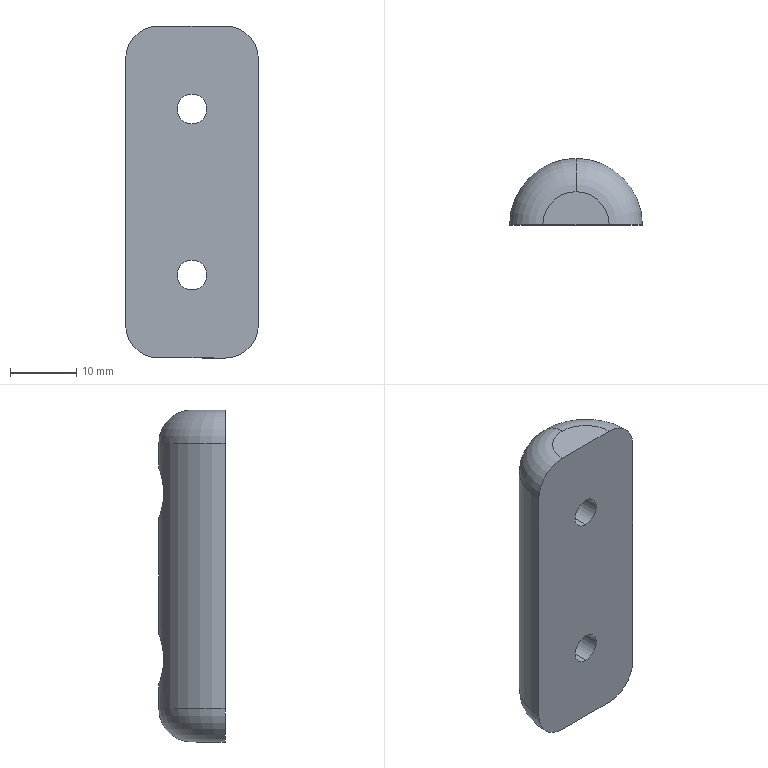Component | SolidWorks | DZ.KX.203-TC1505-30-09-01-05-32-3 | 1 solid | 19 faces | box 20 x 10 x 50 mm | volume 6913 mm3 | cylinder 10 | plane 5 | torus 4 | commonest cylinder face diameters 4.5 x4 7.5 x4 20 x2
build123d program:
from build123d import *

# Parameters (mm, degrees)
BOSS_EXTRUDE1_DEPTH                               = 50
HOLE_SIZE_ACCORDING_TO_HEXAGON_SOCKET_D           = 4.5
HOLE_SIZE_ACCORDING_TO_HEXAGON_SOCKET_CBORE_D     = 7.5
HOLE_SIZE_ACCORDING_TO_HEXAGON_SOCKET_CBORE_DEPTH = 6
FILLET1_R                                         = 5


with BuildPart() as part:
    # Sketch1 → Boss-Extrude1 (new body)
    with BuildSketch(Plane(origin=(0, 0, 0), x_dir=(0, 0, -1), z_dir=(1, 0, 0))):
        with BuildLine():
            Line((0, 10), (0, -10))
            ThreePointArc((0, -10), (-10, 0), (0, 10))
        make_face()
    extrude(amount=BOSS_EXTRUDE1_DEPTH)

    # Hole Size _according to_ Hexagon Socket (through all)
    with Locations(Plane(origin=(10, 0, 10), x_dir=(-1, 0, 0), z_dir=(0, 0, 1))):
        with Locations((-2.5, 0), (-27.5, 0)):
            CounterBoreHole(HOLE_SIZE_ACCORDING_TO_HEXAGON_SOCKET_D / 2, HOLE_SIZE_ACCORDING_TO_HEXAGON_SOCKET_CBORE_D / 2, HOLE_SIZE_ACCORDING_TO_HEXAGON_SOCKET_CBORE_DEPTH)

    # Fillet1
    fillet1_edges = [part.edges().sort_by_distance(p)[0] for p in [
        (0, 0, 10),
        (50, 0, 10),
    ]]
    fillet(fillet1_edges, radius=FILLET1_R)


solid = part.part

# Placed as in the assembly
solid = solid.moved(Location((248.5, -528.807, 17.16), (-90, 0, 90)))
STEP:
#1=COLOUR_RGB('',0.7922,0.8196,0.9333);
#2=FILL_AREA_STYLE_COLOUR('',#1);
#3=FILL_AREA_STYLE('',(#2));
#4=SURFACE_STYLE_FILL_AREA(#3);
#5=SURFACE_SIDE_STYLE('',(#4));
#6=SURFACE_STYLE_USAGE(.BOTH.,#5);
#7=PRESENTATION_STYLE_ASSIGNMENT((#6));
#8=CARTESIAN_POINT('',(9.783,-20.425,-1.096));
#9=VERTEX_POINT('',#8);
#10=CARTESIAN_POINT('',(9.39,-20.819,-1.096));
#11=VERTEX_POINT('',#10);
#12=CARTESIAN_POINT('',(9.783,-20.819,-1.096));
#13=DIRECTION('',(0.,0.,1.));
#14=DIRECTION('',(-0.,-1.,0.));
#15=AXIS2_PLACEMENT_3D('',#12,#13,#14);
#16=CIRCLE('',#15,0.3937);
#17=EDGE_CURVE('',#9,#11,#16,.T.);
#18=ORIENTED_EDGE('',*,*,#17,.F.);
#19=CARTESIAN_POINT('',(9.783,-20.622,-1.293));
#20=VERTEX_POINT('',#19);
#21=CARTESIAN_POINT('',(9.783,-20.622,-1.096));
#22=DIRECTION('',(-1.,0.,0.));
#23=DIRECTION('',(-0.,-1.,0.));
#24=AXIS2_PLACEMENT_3D('',#21,#22,#23);
#25=CIRCLE('',#24,0.1969);
#26=EDGE_CURVE('',#9,#20,#25,.T.);
#27=ORIENTED_EDGE('',*,*,#26,.T.);
#28=CARTESIAN_POINT('',(9.587,-20.819,-1.293));
#29=VERTEX_POINT('',#28);
#30=CARTESIAN_POINT('',(9.783,-20.819,-1.293));
#31=DIRECTION('',(-0.,-0.,-1.));
#32=DIRECTION('',(-0.,-1.,0.));
#33=AXIS2_PLACEMENT_3D('',#30,#31,#32);
#34=CIRCLE('',#33,0.1969);
#35=EDGE_CURVE('',#29,#20,#34,.T.);
#36=ORIENTED_EDGE('',*,*,#35,.F.);
#37=CARTESIAN_POINT('',(9.587,-20.819,-1.096));
#38=DIRECTION('',(-0.,-1.,0.));
#39=DIRECTION('',(-0.,0.,-1.));
#40=AXIS2_PLACEMENT_3D('',#37,#38,#39);
#41=CIRCLE('',#40,0.1969);
#42=EDGE_CURVE('',#11,#29,#41,.T.);
#43=ORIENTED_EDGE('',*,*,#42,.F.);
#44=EDGE_LOOP('',(#18,#27,#36,#43));
#45=FACE_OUTER_BOUND('',#44,.T.);
#46=CARTESIAN_POINT('',(9.783,-20.819,-1.096));
#47=DIRECTION('',(-0.,-0.,-1.));
#48=DIRECTION('',(-0.,-1.,0.));
#49=AXIS2_PLACEMENT_3D('',#46,#47,#48);
#50=TOROIDAL_SURFACE('',#49,0.1969,0.1969);
#51=ADVANCED_FACE('',(#45),#50,.T.);
#52=CARTESIAN_POINT('',(9.783,-20.622,0.6756));
#53=VERTEX_POINT('',#52);
#54=CARTESIAN_POINT('',(9.587,-20.819,0.6756));
#55=VERTEX_POINT('',#54);
#56=CARTESIAN_POINT('',(9.783,-20.819,0.6756));
#57=DIRECTION('',(0.,0.,1.));
#58=DIRECTION('',(-0.,-1.,0.));
#59=AXIS2_PLACEMENT_3D('',#56,#57,#58);
#60=CIRCLE('',#59,0.1969);
#61=EDGE_CURVE('',#53,#55,#60,.T.);
#62=ORIENTED_EDGE('',*,*,#61,.F.);
#63=CARTESIAN_POINT('',(9.783,-20.425,0.4787));
#64=VERTEX_POINT('',#63);
#65=CARTESIAN_POINT('',(9.783,-20.622,0.4787));
#66=DIRECTION('',(-1.,0.,0.));
#67=DIRECTION('',(-0.,-1.,0.));
#68=AXIS2_PLACEMENT_3D('',#65,#66,#67);
#69=CIRCLE('',#68,0.1969);
#70=EDGE_CURVE('',#53,#64,#69,.T.);
#71=ORIENTED_EDGE('',*,*,#70,.T.);
#72=CARTESIAN_POINT('',(9.39,-20.819,0.4787));
#73=VERTEX_POINT('',#72);
#74=CARTESIAN_POINT('',(9.783,-20.819,0.4787));
#75=DIRECTION('',(-0.,-0.,-1.));
#76=DIRECTION('',(-0.,-1.,0.));
#77=AXIS2_PLACEMENT_3D('',#74,#75,#76);
#78=CIRCLE('',#77,0.3937);
#79=EDGE_CURVE('',#73,#64,#78,.T.);
#80=ORIENTED_EDGE('',*,*,#79,.F.);
#81=CARTESIAN_POINT('',(9.587,-20.819,0.4787));
#82=DIRECTION('',(-0.,-1.,0.));
#83=DIRECTION('',(0.,0.,-1.));
#84=AXIS2_PLACEMENT_3D('',#81,#82,#83);
#85=CIRCLE('',#84,0.1969);
#86=EDGE_CURVE('',#55,#73,#85,.T.);
#87=ORIENTED_EDGE('',*,*,#86,.F.);
#88=EDGE_LOOP('',(#62,#71,#80,#87));
#89=FACE_OUTER_BOUND('',#88,.T.);
#90=CARTESIAN_POINT('',(9.783,-20.819,0.4787));
#91=DIRECTION('',(-0.,-0.,-1.));
#92=DIRECTION('',(-0.,-1.,0.));
#93=AXIS2_PLACEMENT_3D('',#90,#91,#92);
#94=TOROIDAL_SURFACE('',#93,0.1969,0.1969);
#95=ADVANCED_FACE('',(#89),#94,.T.);
#96=CARTESIAN_POINT('',(9.783,-20.819,0.272));
#97=VERTEX_POINT('',#96);
#98=CARTESIAN_POINT('',(9.783,-20.819,0.09486));
#99=VERTEX_POINT('',#98);
#100=CARTESIAN_POINT('',(9.783,-20.819,0.1834));
#101=DIRECTION('',(0.,1.,-0.));
#102=DIRECTION('',(0.,0.,-1.));
#103=AXIS2_PLACEMENT_3D('',#100,#101,#102);
#104=CIRCLE('',#103,0.08858);
#105=EDGE_CURVE('',#97,#99,#104,.T.);
#106=ORIENTED_EDGE('',*,*,#105,.F.);
#107=CARTESIAN_POINT('',(9.783,-20.662,0.272));
#108=VERTEX_POINT('',#107);
#109=CARTESIAN_POINT('',(9.783,-20.425,0.272));
#110=DIRECTION('',(0.,1.,-0.));
#111=VECTOR('',#110,39.37);
#112=LINE('',#109,#111);
#113=EDGE_CURVE('',#97,#108,#112,.T.);
#114=ORIENTED_EDGE('',*,*,#113,.T.);
#115=CARTESIAN_POINT('',(9.783,-20.662,0.09486));
#116=VERTEX_POINT('',#115);
#117=CARTESIAN_POINT('',(9.783,-20.662,0.1834));
#118=DIRECTION('',(0.,1.,-0.));
#119=DIRECTION('',(0.,0.,-1.));
#120=AXIS2_PLACEMENT_3D('',#117,#118,#119);
#121=CIRCLE('',#120,0.08858);
#122=EDGE_CURVE('',#108,#116,#121,.T.);
#123=ORIENTED_EDGE('',*,*,#122,.T.);
#124=CARTESIAN_POINT('',(9.783,-20.425,0.09486));
#125=DIRECTION('',(0.,1.,-0.));
#126=VECTOR('',#125,39.37);
#127=LINE('',#124,#126);
#128=EDGE_CURVE('',#99,#116,#127,.T.);
#129=ORIENTED_EDGE('',*,*,#128,.F.);
#130=EDGE_LOOP('',(#106,#114,#123,#129));
#131=FACE_OUTER_BOUND('',#130,.T.);
#132=CARTESIAN_POINT('',(9.783,-20.425,0.1834));
#133=DIRECTION('',(0.,1.,-0.));
#134=DIRECTION('',(0.,0.,-1.));
#135=AXIS2_PLACEMENT_3D('',#132,#133,#134);
#136=CYLINDRICAL_SURFACE('',#135,0.08858);
#137=ADVANCED_FACE('',(#131),#136,.F.);
#138=CARTESIAN_POINT('',(9.783,-20.662,0.3311));
#139=VERTEX_POINT('',#138);
#140=CARTESIAN_POINT('',(9.783,-20.662,0.03581));
#141=VERTEX_POINT('',#140);
#142=CARTESIAN_POINT('',(9.783,-20.662,0.1834));
#143=DIRECTION('',(0.,1.,-0.));
#144=DIRECTION('',(0.,0.,-1.));
#145=AXIS2_PLACEMENT_3D('',#142,#143,#144);
#146=CIRCLE('',#145,0.1476);
#147=EDGE_CURVE('',#139,#141,#146,.T.);
#148=ORIENTED_EDGE('',*,*,#147,.F.);
#149=CARTESIAN_POINT('',(9.783,-20.425,0.3311));
#150=VERTEX_POINT('',#149);
#151=CARTESIAN_POINT('',(9.783,-20.425,0.3311));
#152=DIRECTION('',(0.,1.,-0.));
#153=VECTOR('',#152,39.37);
#154=LINE('',#151,#153);
#155=EDGE_CURVE('',#139,#150,#154,.T.);
#156=ORIENTED_EDGE('',*,*,#155,.T.);
#157=CARTESIAN_POINT('',(9.783,-20.425,0.03581));
#158=VERTEX_POINT('',#157);
#159=CARTESIAN_POINT('',(9.783,-20.425,0.03581));
#160=CARTESIAN_POINT('',(9.793,-20.425,0.03581));
#161=CARTESIAN_POINT('',(9.803,-20.426,0.03679));
#162=CARTESIAN_POINT('',(9.822,-20.427,0.04059));
#163=CARTESIAN_POINT('',(9.831,-20.428,0.04348));
#164=CARTESIAN_POINT('',(9.849,-20.431,0.05093));
#165=CARTESIAN_POINT('',(9.858,-20.432,0.05547));
#166=CARTESIAN_POINT('',(9.874,-20.436,0.06619));
#167=CARTESIAN_POINT('',(9.881,-20.438,0.07236));
#168=CARTESIAN_POINT('',(9.895,-20.441,0.08586));
#169=CARTESIAN_POINT('',(9.901,-20.443,0.09325));
#170=CARTESIAN_POINT('',(9.912,-20.447,0.1093));
#171=CARTESIAN_POINT('',(9.916,-20.448,0.1178));
#172=CARTESIAN_POINT('',(9.923,-20.451,0.1355));
#173=CARTESIAN_POINT('',(9.926,-20.452,0.1449));
#174=CARTESIAN_POINT('',(9.93,-20.454,0.164));
#175=CARTESIAN_POINT('',(9.931,-20.454,0.1736));
#176=CARTESIAN_POINT('',(9.931,-20.454,0.1931));
#177=CARTESIAN_POINT('',(9.93,-20.454,0.203));
#178=CARTESIAN_POINT('',(9.926,-20.452,0.222));
#179=CARTESIAN_POINT('',(9.923,-20.451,0.2312));
#180=CARTESIAN_POINT('',(9.916,-20.448,0.2492));
#181=CARTESIAN_POINT('',(9.911,-20.447,0.2577));
#182=CARTESIAN_POINT('',(9.901,-20.443,0.2736));
#183=CARTESIAN_POINT('',(9.895,-20.441,0.2811));
#184=CARTESIAN_POINT('',(9.881,-20.438,0.2947));
#185=CARTESIAN_POINT('',(9.874,-20.436,0.3007));
#186=CARTESIAN_POINT('',(9.858,-20.432,0.3114));
#187=CARTESIAN_POINT('',(9.849,-20.431,0.316));
#188=CARTESIAN_POINT('',(9.831,-20.428,0.3234));
#189=CARTESIAN_POINT('',(9.822,-20.427,0.3263));
#190=CARTESIAN_POINT('',(9.803,-20.426,0.3301));
#191=CARTESIAN_POINT('',(9.793,-20.425,0.3311));
#192=CARTESIAN_POINT('',(9.783,-20.425,0.3311));
#193=B_SPLINE_CURVE_WITH_KNOTS('',3,(#159,#160,#161,#162,#163,#164,#165,#166,#167,#168,#169,#170,#171,#172,#173,#174,#175,#176,#177,#178,#179,#180,#181,#182,#183,#184,#185,#186,#187,#188,#189,#190,#191,#192),.UNSPECIFIED.,.F.,.F.,(4,2,2,2,2,2,2,2,2,2,2,2,2,2,2,2,4),(0.,0.0007396,0.001479,0.002219,0.002958,0.003698,0.004438,0.005177,0.005917,0.006656,0.007396,0.008135,0.008875,0.009615,0.01035,0.01109,0.01183),.UNSPECIFIED.);
#194=EDGE_CURVE('',#158,#150,#193,.T.);
#195=ORIENTED_EDGE('',*,*,#194,.F.);
#196=CARTESIAN_POINT('',(9.783,-20.425,0.03581));
#197=DIRECTION('',(0.,1.,-0.));
#198=VECTOR('',#197,39.37);
#199=LINE('',#196,#198);
#200=EDGE_CURVE('',#141,#158,#199,.T.);
#201=ORIENTED_EDGE('',*,*,#200,.F.);
#202=EDGE_LOOP('',(#148,#156,#195,#201));
#203=FACE_OUTER_BOUND('',#202,.T.);
#204=CARTESIAN_POINT('',(9.783,-20.425,0.1834));
#205=DIRECTION('',(0.,1.,-0.));
#206=DIRECTION('',(0.,0.,-1.));
#207=AXIS2_PLACEMENT_3D('',#204,#205,#206);
#208=CYLINDRICAL_SURFACE('',#207,0.1476);
#209=ADVANCED_FACE('',(#203),#208,.F.);
#210=CARTESIAN_POINT('',(9.783,-20.819,-0.7122));
#211=VERTEX_POINT('',#210);
#212=CARTESIAN_POINT('',(9.783,-20.819,-0.8894));
#213=VERTEX_POINT('',#212);
#214=CARTESIAN_POINT('',(9.783,-20.819,-0.8008));
#215=DIRECTION('',(0.,1.,-0.));
#216=DIRECTION('',(0.,0.,-1.));
#217=AXIS2_PLACEMENT_3D('',#214,#215,#216);
#218=CIRCLE('',#217,0.08858);
#219=EDGE_CURVE('',#211,#213,#218,.T.);
#220=ORIENTED_EDGE('',*,*,#219,.F.);
#221=CARTESIAN_POINT('',(9.783,-20.662,-0.7122));
#222=VERTEX_POINT('',#221);
#223=CARTESIAN_POINT('',(9.783,-20.425,-0.7122));
#224=DIRECTION('',(0.,1.,-0.));
#225=VECTOR('',#224,39.37);
#226=LINE('',#223,#225);
#227=EDGE_CURVE('',#211,#222,#226,.T.);
#228=ORIENTED_EDGE('',*,*,#227,.T.);
#229=CARTESIAN_POINT('',(9.783,-20.662,-0.8894));
#230=VERTEX_POINT('',#229);
#231=CARTESIAN_POINT('',(9.783,-20.662,-0.8008));
#232=DIRECTION('',(0.,1.,-0.));
#233=DIRECTION('',(0.,0.,-1.));
#234=AXIS2_PLACEMENT_3D('',#231,#232,#233);
#235=CIRCLE('',#234,0.08858);
#236=EDGE_CURVE('',#222,#230,#235,.T.);
#237=ORIENTED_EDGE('',*,*,#236,.T.);
#238=CARTESIAN_POINT('',(9.783,-20.425,-0.8894));
#239=DIRECTION('',(0.,1.,-0.));
#240=VECTOR('',#239,39.37);
#241=LINE('',#238,#240);
#242=EDGE_CURVE('',#213,#230,#241,.T.);
#243=ORIENTED_EDGE('',*,*,#242,.F.);
#244=EDGE_LOOP('',(#220,#228,#237,#243));
#245=FACE_OUTER_BOUND('',#244,.T.);
#246=CARTESIAN_POINT('',(9.783,-20.425,-0.8008));
#247=DIRECTION('',(0.,1.,-0.));
#248=DIRECTION('',(0.,0.,-1.));
#249=AXIS2_PLACEMENT_3D('',#246,#247,#248);
#250=CYLINDRICAL_SURFACE('',#249,0.08858);
#251=ADVANCED_FACE('',(#245),#250,.F.);
#252=CARTESIAN_POINT('',(9.783,-20.662,-0.6532));
#253=VERTEX_POINT('',#252);
#254=CARTESIAN_POINT('',(9.783,-20.662,-0.9484));
#255=VERTEX_POINT('',#254);
#256=CARTESIAN_POINT('',(9.783,-20.662,-0.8008));
#257=DIRECTION('',(0.,1.,-0.));
#258=DIRECTION('',(0.,0.,-1.));
#259=AXIS2_PLACEMENT_3D('',#256,#257,#258);
#260=CIRCLE('',#259,0.1476);
#261=EDGE_CURVE('',#253,#255,#260,.T.);
#262=ORIENTED_EDGE('',*,*,#261,.F.);
#263=CARTESIAN_POINT('',(9.783,-20.425,-0.6532));
#264=VERTEX_POINT('',#263);
#265=CARTESIAN_POINT('',(9.783,-20.425,-0.6532));
#266=DIRECTION('',(0.,1.,-0.));
#267=VECTOR('',#266,39.37);
#268=LINE('',#265,#267);
#269=EDGE_CURVE('',#253,#264,#268,.T.);
#270=ORIENTED_EDGE('',*,*,#269,.T.);
#271=CARTESIAN_POINT('',(9.783,-20.425,-0.9484));
#272=VERTEX_POINT('',#271);
#273=CARTESIAN_POINT('',(9.783,-20.425,-0.9484));
#274=CARTESIAN_POINT('',(9.793,-20.425,-0.9484));
#275=CARTESIAN_POINT('',(9.803,-20.426,-0.9475));
#276=CARTESIAN_POINT('',(9.822,-20.427,-0.9437));
#277=CARTESIAN_POINT('',(9.831,-20.428,-0.9408));
#278=CARTESIAN_POINT('',(9.849,-20.431,-0.9333));
#279=CARTESIAN_POINT('',(9.858,-20.432,-0.9288));
#280=CARTESIAN_POINT('',(9.874,-20.436,-0.9181));
#281=CARTESIAN_POINT('',(9.881,-20.438,-0.9119));
#282=CARTESIAN_POINT('',(9.895,-20.441,-0.8984));
#283=CARTESIAN_POINT('',(9.901,-20.443,-0.891));
#284=CARTESIAN_POINT('',(9.912,-20.447,-0.8749));
#285=CARTESIAN_POINT('',(9.916,-20.448,-0.8665));
#286=CARTESIAN_POINT('',(9.923,-20.451,-0.8488));
#287=CARTESIAN_POINT('',(9.926,-20.452,-0.8394));
#288=CARTESIAN_POINT('',(9.93,-20.454,-0.8203));
#289=CARTESIAN_POINT('',(9.931,-20.454,-0.8106));
#290=CARTESIAN_POINT('',(9.931,-20.454,-0.7912));
#291=CARTESIAN_POINT('',(9.93,-20.454,-0.7813));
#292=CARTESIAN_POINT('',(9.926,-20.452,-0.7623));
#293=CARTESIAN_POINT('',(9.923,-20.451,-0.753));
#294=CARTESIAN_POINT('',(9.916,-20.448,-0.735));
#295=CARTESIAN_POINT('',(9.911,-20.447,-0.7265));
#296=CARTESIAN_POINT('',(9.901,-20.443,-0.7106));
#297=CARTESIAN_POINT('',(9.895,-20.441,-0.7031));
#298=CARTESIAN_POINT('',(9.881,-20.438,-0.6896));
#299=CARTESIAN_POINT('',(9.874,-20.436,-0.6835));
#300=CARTESIAN_POINT('',(9.858,-20.432,-0.6728));
#301=CARTESIAN_POINT('',(9.849,-20.431,-0.6682));
#302=CARTESIAN_POINT('',(9.831,-20.428,-0.6608));
#303=CARTESIAN_POINT('',(9.822,-20.427,-0.658));
#304=CARTESIAN_POINT('',(9.803,-20.426,-0.6541));
#305=CARTESIAN_POINT('',(9.793,-20.425,-0.6532));
#306=CARTESIAN_POINT('',(9.783,-20.425,-0.6532));
#307=B_SPLINE_CURVE_WITH_KNOTS('',3,(#273,#274,#275,#276,#277,#278,#279,#280,#281,#282,#283,#284,#285,#286,#287,#288,#289,#290,#291,#292,#293,#294,#295,#296,#297,#298,#299,#300,#301,#302,#303,#304,#305,#306),.UNSPECIFIED.,.F.,.F.,(4,2,2,2,2,2,2,2,2,2,2,2,2,2,2,2,4),(0.,0.0007396,0.001479,0.002219,0.002958,0.003698,0.004438,0.005177,0.005917,0.006656,0.007396,0.008135,0.008875,0.009615,0.01035,0.01109,0.01183),.UNSPECIFIED.);
#308=EDGE_CURVE('',#272,#264,#307,.T.);
#309=ORIENTED_EDGE('',*,*,#308,.F.);
#310=CARTESIAN_POINT('',(9.783,-20.425,-0.9484));
#311=DIRECTION('',(0.,1.,-0.));
#312=VECTOR('',#311,39.37);
#313=LINE('',#310,#312);
#314=EDGE_CURVE('',#255,#272,#313,.T.);
#315=ORIENTED_EDGE('',*,*,#314,.F.);
#316=EDGE_LOOP('',(#262,#270,#309,#315));
#317=FACE_OUTER_BOUND('',#316,.T.);
#318=CARTESIAN_POINT('',(9.783,-20.425,-0.8008));
#319=DIRECTION('',(0.,1.,-0.));
#320=DIRECTION('',(0.,0.,-1.));
#321=AXIS2_PLACEMENT_3D('',#318,#319,#320);
#322=CYLINDRICAL_SURFACE('',#321,0.1476);
#323=ADVANCED_FACE('',(#317),#322,.F.);
#324=CARTESIAN_POINT('',(10.177,-20.819,-1.096));
#325=VERTEX_POINT('',#324);
#326=CARTESIAN_POINT('',(9.783,-20.819,-1.096));
#327=DIRECTION('',(0.,0.,1.));
#328=DIRECTION('',(-0.,-1.,0.));
#329=AXIS2_PLACEMENT_3D('',#326,#327,#328);
#330=CIRCLE('',#329,0.3937);
#331=EDGE_CURVE('',#325,#9,#330,.T.);
#332=ORIENTED_EDGE('',*,*,#331,.T.);
#333=CARTESIAN_POINT('',(9.783,-20.425,-1.293));
#334=DIRECTION('',(0.,0.,1.));
#335=VECTOR('',#334,39.37);
#336=LINE('',#333,#335);
#337=EDGE_CURVE('',#9,#272,#336,.T.);
#338=ORIENTED_EDGE('',*,*,#337,.T.);
#339=ORIENTED_EDGE('',*,*,#308,.T.);
#340=CARTESIAN_POINT('',(9.783,-20.425,-1.293));
#341=DIRECTION('',(0.,0.,1.));
#342=VECTOR('',#341,39.37);
#343=LINE('',#340,#342);
#344=EDGE_CURVE('',#264,#158,#343,.T.);
#345=ORIENTED_EDGE('',*,*,#344,.T.);
#346=ORIENTED_EDGE('',*,*,#194,.T.);
#347=CARTESIAN_POINT('',(9.783,-20.425,-1.293));
#348=DIRECTION('',(0.,0.,1.));
#349=VECTOR('',#348,39.37);
#350=LINE('',#347,#349);
#351=EDGE_CURVE('',#150,#64,#350,.T.);
#352=ORIENTED_EDGE('',*,*,#351,.T.);
#353=CARTESIAN_POINT('',(10.177,-20.819,0.4787));
#354=VERTEX_POINT('',#353);
#355=CARTESIAN_POINT('',(9.783,-20.819,0.4787));
#356=DIRECTION('',(-0.,-0.,-1.));
#357=DIRECTION('',(-0.,-1.,0.));
#358=AXIS2_PLACEMENT_3D('',#355,#356,#357);
#359=CIRCLE('',#358,0.3937);
#360=EDGE_CURVE('',#64,#354,#359,.T.);
#361=ORIENTED_EDGE('',*,*,#360,.T.);
#362=CARTESIAN_POINT('',(10.177,-20.819,-1.293));
#363=DIRECTION('',(0.,0.,1.));
#364=VECTOR('',#363,39.37);
#365=LINE('',#362,#364);
#366=EDGE_CURVE('',#325,#354,#365,.T.);
#367=ORIENTED_EDGE('',*,*,#366,.F.);
#368=EDGE_LOOP('',(#332,#338,#339,#345,#346,#352,#361,#367));
#369=FACE_OUTER_BOUND('',#368,.T.);
#370=CARTESIAN_POINT('',(9.783,-20.819,-1.293));
#371=DIRECTION('',(0.,0.,1.));
#372=DIRECTION('',(0.,1.,-0.));
#373=AXIS2_PLACEMENT_3D('',#370,#371,#372);
#374=CYLINDRICAL_SURFACE('',#373,0.3937);
#375=ADVANCED_FACE('',(#369),#374,.T.);
#376=ORIENTED_EDGE('',*,*,#337,.F.);
#377=ORIENTED_EDGE('',*,*,#17,.T.);
#378=CARTESIAN_POINT('',(9.39,-20.819,-1.293));
#379=DIRECTION('',(0.,0.,1.));
#380=VECTOR('',#379,39.37);
#381=LINE('',#378,#380);
#382=EDGE_CURVE('',#11,#73,#381,.T.);
#383=ORIENTED_EDGE('',*,*,#382,.T.);
#384=ORIENTED_EDGE('',*,*,#79,.T.);
#385=ORIENTED_EDGE('',*,*,#351,.F.);
#386=CARTESIAN_POINT('',(9.783,-20.425,0.3311));
#387=CARTESIAN_POINT('',(9.774,-20.425,0.3311));
#388=CARTESIAN_POINT('',(9.764,-20.426,0.3301));
#389=CARTESIAN_POINT('',(9.745,-20.427,0.3263));
#390=CARTESIAN_POINT('',(9.736,-20.428,0.3234));
#391=CARTESIAN_POINT('',(9.718,-20.431,0.316));
#392=CARTESIAN_POINT('',(9.709,-20.432,0.3114));
#393=CARTESIAN_POINT('',(9.693,-20.436,0.3007));
#394=CARTESIAN_POINT('',(9.686,-20.438,0.2946));
#395=CARTESIAN_POINT('',(9.672,-20.441,0.2809));
#396=CARTESIAN_POINT('',(9.666,-20.443,0.2735));
#397=CARTESIAN_POINT('',(9.655,-20.447,0.2577));
#398=CARTESIAN_POINT('',(9.651,-20.448,0.2491));
#399=CARTESIAN_POINT('',(9.643,-20.451,0.2312));
#400=CARTESIAN_POINT('',(9.641,-20.452,0.222));
#401=CARTESIAN_POINT('',(9.637,-20.454,0.203));
#402=CARTESIAN_POINT('',(9.636,-20.454,0.1931));
#403=CARTESIAN_POINT('',(9.636,-20.454,0.1737));
#404=CARTESIAN_POINT('',(9.637,-20.454,0.164));
#405=CARTESIAN_POINT('',(9.641,-20.452,0.1448));
#406=CARTESIAN_POINT('',(9.644,-20.451,0.1355));
#407=CARTESIAN_POINT('',(9.651,-20.448,0.1177));
#408=CARTESIAN_POINT('',(9.656,-20.447,0.1091));
#409=CARTESIAN_POINT('',(9.666,-20.443,0.09315));
#410=CARTESIAN_POINT('',(9.672,-20.441,0.08579));
#411=CARTESIAN_POINT('',(9.686,-20.438,0.07225));
#412=CARTESIAN_POINT('',(9.693,-20.436,0.06607));
#413=CARTESIAN_POINT('',(9.709,-20.432,0.05543));
#414=CARTESIAN_POINT('',(9.718,-20.431,0.05089));
#415=CARTESIAN_POINT('',(9.736,-20.428,0.04342));
#416=CARTESIAN_POINT('',(9.745,-20.427,0.04057));
#417=CARTESIAN_POINT('',(9.764,-20.426,0.03679));
#418=CARTESIAN_POINT('',(9.774,-20.425,0.03581));
#419=CARTESIAN_POINT('',(9.783,-20.425,0.03581));
#420=B_SPLINE_CURVE_WITH_KNOTS('',3,(#386,#387,#388,#389,#390,#391,#392,#393,#394,#395,#396,#397,#398,#399,#400,#401,#402,#403,#404,#405,#406,#407,#408,#409,#410,#411,#412,#413,#414,#415,#416,#417,#418,#419),.UNSPECIFIED.,.F.,.F.,(4,2,2,2,2,2,2,2,2,2,2,2,2,2,2,2,4),(0.01183,0.01257,0.01331,0.01405,0.01479,0.01553,0.01627,0.01701,0.01775,0.01849,0.01923,0.01997,0.02071,0.02145,0.02219,0.02292,0.02366),.UNSPECIFIED.);
#421=EDGE_CURVE('',#150,#158,#420,.T.);
#422=ORIENTED_EDGE('',*,*,#421,.T.);
#423=ORIENTED_EDGE('',*,*,#344,.F.);
#424=CARTESIAN_POINT('',(9.783,-20.425,-0.6532));
#425=CARTESIAN_POINT('',(9.774,-20.425,-0.6532));
#426=CARTESIAN_POINT('',(9.764,-20.426,-0.6541));
#427=CARTESIAN_POINT('',(9.745,-20.427,-0.658));
#428=CARTESIAN_POINT('',(9.736,-20.428,-0.6608));
#429=CARTESIAN_POINT('',(9.718,-20.431,-0.6683));
#430=CARTESIAN_POINT('',(9.709,-20.432,-0.6729));
#431=CARTESIAN_POINT('',(9.693,-20.436,-0.6836));
#432=CARTESIAN_POINT('',(9.686,-20.438,-0.6897));
#433=CARTESIAN_POINT('',(9.672,-20.441,-0.7033));
#434=CARTESIAN_POINT('',(9.666,-20.443,-0.7107));
#435=CARTESIAN_POINT('',(9.655,-20.447,-0.7266));
#436=CARTESIAN_POINT('',(9.651,-20.448,-0.7352));
#437=CARTESIAN_POINT('',(9.643,-20.451,-0.753));
#438=CARTESIAN_POINT('',(9.641,-20.452,-0.7623));
#439=CARTESIAN_POINT('',(9.637,-20.454,-0.7812));
#440=CARTESIAN_POINT('',(9.636,-20.454,-0.7911));
#441=CARTESIAN_POINT('',(9.636,-20.454,-0.8106));
#442=CARTESIAN_POINT('',(9.637,-20.454,-0.8203));
#443=CARTESIAN_POINT('',(9.641,-20.452,-0.8394));
#444=CARTESIAN_POINT('',(9.644,-20.451,-0.8488));
#445=CARTESIAN_POINT('',(9.651,-20.448,-0.8665));
#446=CARTESIAN_POINT('',(9.656,-20.447,-0.8751));
#447=CARTESIAN_POINT('',(9.666,-20.443,-0.8911));
#448=CARTESIAN_POINT('',(9.672,-20.441,-0.8985));
#449=CARTESIAN_POINT('',(9.686,-20.438,-0.912));
#450=CARTESIAN_POINT('',(9.693,-20.436,-0.9182));
#451=CARTESIAN_POINT('',(9.709,-20.432,-0.9288));
#452=CARTESIAN_POINT('',(9.718,-20.431,-0.9334));
#453=CARTESIAN_POINT('',(9.736,-20.428,-0.9408));
#454=CARTESIAN_POINT('',(9.745,-20.427,-0.9437));
#455=CARTESIAN_POINT('',(9.764,-20.426,-0.9475));
#456=CARTESIAN_POINT('',(9.774,-20.425,-0.9484));
#457=CARTESIAN_POINT('',(9.783,-20.425,-0.9484));
#458=B_SPLINE_CURVE_WITH_KNOTS('',3,(#424,#425,#426,#427,#428,#429,#430,#431,#432,#433,#434,#435,#436,#437,#438,#439,#440,#441,#442,#443,#444,#445,#446,#447,#448,#449,#450,#451,#452,#453,#454,#455,#456,#457),.UNSPECIFIED.,.F.,.F.,(4,2,2,2,2,2,2,2,2,2,2,2,2,2,2,2,4),(0.01183,0.01257,0.01331,0.01405,0.01479,0.01553,0.01627,0.01701,0.01775,0.01849,0.01923,0.01997,0.02071,0.02145,0.02219,0.02292,0.02366),.UNSPECIFIED.);
#459=EDGE_CURVE('',#264,#272,#458,.T.);
#460=ORIENTED_EDGE('',*,*,#459,.T.);
#461=EDGE_LOOP('',(#376,#377,#383,#384,#385,#422,#423,#460));
#462=FACE_OUTER_BOUND('',#461,.T.);
#463=CARTESIAN_POINT('',(9.783,-20.819,-1.293));
#464=DIRECTION('',(0.,0.,1.));
#465=DIRECTION('',(0.,1.,-0.));
#466=AXIS2_PLACEMENT_3D('',#463,#464,#465);
#467=CYLINDRICAL_SURFACE('',#466,0.3937);
#468=ADVANCED_FACE('',(#462),#467,.T.);
#469=CARTESIAN_POINT('',(9.783,-20.819,0.1834));
#470=DIRECTION('',(0.,1.,-0.));
#471=DIRECTION('',(0.,0.,-1.));
#472=AXIS2_PLACEMENT_3D('',#469,#470,#471);
#473=CIRCLE('',#472,0.08858);
#474=EDGE_CURVE('',#99,#97,#473,.T.);
#475=ORIENTED_EDGE('',*,*,#474,.T.);
#476=ORIENTED_EDGE('',*,*,#105,.T.);
#477=EDGE_LOOP('',(#475,#476));
#478=FACE_BOUND('',#477,.T.);
#479=CARTESIAN_POINT('',(9.783,-20.819,-0.8008));
#480=DIRECTION('',(0.,1.,-0.));
#481=DIRECTION('',(0.,0.,-1.));
#482=AXIS2_PLACEMENT_3D('',#479,#480,#481);
#483=CIRCLE('',#482,0.08858);
#484=EDGE_CURVE('',#213,#211,#483,.T.);
#485=ORIENTED_EDGE('',*,*,#484,.T.);
#486=ORIENTED_EDGE('',*,*,#219,.T.);
#487=EDGE_LOOP('',(#485,#486));
#488=FACE_BOUND('',#487,.T.);
#489=ORIENTED_EDGE('',*,*,#366,.T.);
#490=CARTESIAN_POINT('',(9.98,-20.819,0.6756));
#491=VERTEX_POINT('',#490);
#492=CARTESIAN_POINT('',(9.98,-20.819,0.4787));
#493=DIRECTION('',(-0.,-1.,0.));
#494=DIRECTION('',(0.,0.,-1.));
#495=AXIS2_PLACEMENT_3D('',#492,#493,#494);
#496=CIRCLE('',#495,0.1969);
#497=EDGE_CURVE('',#354,#491,#496,.T.);
#498=ORIENTED_EDGE('',*,*,#497,.T.);
#499=CARTESIAN_POINT('',(9.39,-20.819,0.6756));
#500=DIRECTION('',(-1.,0.,0.));
#501=VECTOR('',#500,39.37);
#502=LINE('',#499,#501);
#503=EDGE_CURVE('',#491,#55,#502,.T.);
#504=ORIENTED_EDGE('',*,*,#503,.T.);
#505=ORIENTED_EDGE('',*,*,#86,.T.);
#506=ORIENTED_EDGE('',*,*,#382,.F.);
#507=ORIENTED_EDGE('',*,*,#42,.T.);
#508=CARTESIAN_POINT('',(9.98,-20.819,-1.293));
#509=VERTEX_POINT('',#508);
#510=CARTESIAN_POINT('',(9.39,-20.819,-1.293));
#511=DIRECTION('',(-1.,0.,0.));
#512=VECTOR('',#511,39.37);
#513=LINE('',#510,#512);
#514=EDGE_CURVE('',#509,#29,#513,.T.);
#515=ORIENTED_EDGE('',*,*,#514,.F.);
#516=CARTESIAN_POINT('',(9.98,-20.819,-1.096));
#517=DIRECTION('',(-0.,-1.,0.));
#518=DIRECTION('',(0.,0.,-1.));
#519=AXIS2_PLACEMENT_3D('',#516,#517,#518);
#520=CIRCLE('',#519,0.1969);
#521=EDGE_CURVE('',#509,#325,#520,.T.);
#522=ORIENTED_EDGE('',*,*,#521,.T.);
#523=EDGE_LOOP('',(#489,#498,#504,#505,#506,#507,#515,#522));
#524=FACE_OUTER_BOUND('',#523,.T.);
#525=CARTESIAN_POINT('',(9.39,-20.819,-1.293));
#526=DIRECTION('',(0.,1.,-0.));
#527=DIRECTION('',(-0.,-0.,-1.));
#528=AXIS2_PLACEMENT_3D('',#525,#526,#527);
#529=PLANE('',#528);
#530=ADVANCED_FACE('',(#478,#488,#524),#529,.F.);
#531=ORIENTED_EDGE('',*,*,#514,.T.);
#532=ORIENTED_EDGE('',*,*,#35,.T.);
#533=CARTESIAN_POINT('',(9.783,-20.819,-1.293));
#534=DIRECTION('',(-0.,-0.,-1.));
#535=DIRECTION('',(-0.,-1.,0.));
#536=AXIS2_PLACEMENT_3D('',#533,#534,#535);
#537=CIRCLE('',#536,0.1969);
#538=EDGE_CURVE('',#20,#509,#537,.T.);
#539=ORIENTED_EDGE('',*,*,#538,.T.);
#540=EDGE_LOOP('',(#531,#532,#539));
#541=FACE_OUTER_BOUND('',#540,.T.);
#542=CARTESIAN_POINT('',(9.783,-20.819,-1.293));
#543=DIRECTION('',(-0.,-0.,-1.));
#544=DIRECTION('',(-0.,-1.,0.));
#545=AXIS2_PLACEMENT_3D('',#542,#543,#544);
#546=PLANE('',#545);
#547=ADVANCED_FACE('',(#541),#546,.T.);
#548=ORIENTED_EDGE('',*,*,#503,.F.);
#549=CARTESIAN_POINT('',(9.783,-20.819,0.6756));
#550=DIRECTION('',(0.,0.,1.));
#551=DIRECTION('',(-0.,-1.,0.));
#552=AXIS2_PLACEMENT_3D('',#549,#550,#551);
#553=CIRCLE('',#552,0.1969);
#554=EDGE_CURVE('',#491,#53,#553,.T.);
#555=ORIENTED_EDGE('',*,*,#554,.T.);
#556=ORIENTED_EDGE('',*,*,#61,.T.);
#557=EDGE_LOOP('',(#548,#555,#556));
#558=FACE_OUTER_BOUND('',#557,.T.);
#559=CARTESIAN_POINT('',(9.783,-20.819,0.6756));
#560=DIRECTION('',(-0.,-0.,-1.));
#561=DIRECTION('',(-0.,-1.,0.));
#562=AXIS2_PLACEMENT_3D('',#559,#560,#561);
#563=PLANE('',#562);
#564=ADVANCED_FACE('',(#558),#563,.F.);
#565=ORIENTED_EDGE('',*,*,#269,.F.);
#566=CARTESIAN_POINT('',(9.783,-20.662,-0.8008));
#567=DIRECTION('',(0.,1.,-0.));
#568=DIRECTION('',(0.,0.,-1.));
#569=AXIS2_PLACEMENT_3D('',#566,#567,#568);
#570=CIRCLE('',#569,0.1476);
#571=EDGE_CURVE('',#255,#253,#570,.T.);
#572=ORIENTED_EDGE('',*,*,#571,.F.);
#573=ORIENTED_EDGE('',*,*,#314,.T.);
#574=ORIENTED_EDGE('',*,*,#459,.F.);
#575=EDGE_LOOP('',(#565,#572,#573,#574));
#576=FACE_OUTER_BOUND('',#575,.T.);
#577=CARTESIAN_POINT('',(9.783,-20.425,-0.8008));
#578=DIRECTION('',(0.,1.,-0.));
#579=DIRECTION('',(0.,0.,-1.));
#580=AXIS2_PLACEMENT_3D('',#577,#578,#579);
#581=CYLINDRICAL_SURFACE('',#580,0.1476);
#582=ADVANCED_FACE('',(#576),#581,.F.);
#583=ORIENTED_EDGE('',*,*,#227,.F.);
#584=ORIENTED_EDGE('',*,*,#484,.F.);
#585=ORIENTED_EDGE('',*,*,#242,.T.);
#586=CARTESIAN_POINT('',(9.783,-20.662,-0.8008));
#587=DIRECTION('',(0.,1.,-0.));
#588=DIRECTION('',(0.,0.,-1.));
#589=AXIS2_PLACEMENT_3D('',#586,#587,#588);
#590=CIRCLE('',#589,0.08858);
#591=EDGE_CURVE('',#230,#222,#590,.T.);
#592=ORIENTED_EDGE('',*,*,#591,.T.);
#593=EDGE_LOOP('',(#583,#584,#585,#592));
#594=FACE_OUTER_BOUND('',#593,.T.);
#595=CARTESIAN_POINT('',(9.783,-20.425,-0.8008));
#596=DIRECTION('',(0.,1.,-0.));
#597=DIRECTION('',(0.,0.,-1.));
#598=AXIS2_PLACEMENT_3D('',#595,#596,#597);
#599=CYLINDRICAL_SURFACE('',#598,0.08858);
#600=ADVANCED_FACE('',(#594),#599,.F.);
#601=ORIENTED_EDGE('',*,*,#591,.F.);
#602=ORIENTED_EDGE('',*,*,#236,.F.);
#603=EDGE_LOOP('',(#601,#602));
#604=FACE_BOUND('',#603,.T.);
#605=ORIENTED_EDGE('',*,*,#571,.T.);
#606=ORIENTED_EDGE('',*,*,#261,.T.);
#607=EDGE_LOOP('',(#605,#606));
#608=FACE_OUTER_BOUND('',#607,.T.);
#609=CARTESIAN_POINT('',(9.783,-20.662,-0.8894));
#610=DIRECTION('',(-0.,-1.,0.));
#611=DIRECTION('',(0.,0.,1.));
#612=AXIS2_PLACEMENT_3D('',#609,#610,#611);
#613=PLANE('',#612);
#614=ADVANCED_FACE('',(#604,#608),#613,.F.);
#615=ORIENTED_EDGE('',*,*,#155,.F.);
#616=CARTESIAN_POINT('',(9.783,-20.662,0.1834));
#617=DIRECTION('',(0.,1.,-0.));
#618=DIRECTION('',(0.,0.,-1.));
#619=AXIS2_PLACEMENT_3D('',#616,#617,#618);
#620=CIRCLE('',#619,0.1476);
#621=EDGE_CURVE('',#141,#139,#620,.T.);
#622=ORIENTED_EDGE('',*,*,#621,.F.);
#623=ORIENTED_EDGE('',*,*,#200,.T.);
#624=ORIENTED_EDGE('',*,*,#421,.F.);
#625=EDGE_LOOP('',(#615,#622,#623,#624));
#626=FACE_OUTER_BOUND('',#625,.T.);
#627=CARTESIAN_POINT('',(9.783,-20.425,0.1834));
#628=DIRECTION('',(0.,1.,-0.));
#629=DIRECTION('',(0.,0.,-1.));
#630=AXIS2_PLACEMENT_3D('',#627,#628,#629);
#631=CYLINDRICAL_SURFACE('',#630,0.1476);
#632=ADVANCED_FACE('',(#626),#631,.F.);
#633=ORIENTED_EDGE('',*,*,#113,.F.);
#634=ORIENTED_EDGE('',*,*,#474,.F.);
#635=ORIENTED_EDGE('',*,*,#128,.T.);
#636=CARTESIAN_POINT('',(9.783,-20.662,0.1834));
#637=DIRECTION('',(0.,1.,-0.));
#638=DIRECTION('',(0.,0.,-1.));
#639=AXIS2_PLACEMENT_3D('',#636,#637,#638);
#640=CIRCLE('',#639,0.08858);
#641=EDGE_CURVE('',#116,#108,#640,.T.);
#642=ORIENTED_EDGE('',*,*,#641,.T.);
#643=EDGE_LOOP('',(#633,#634,#635,#642));
#644=FACE_OUTER_BOUND('',#643,.T.);
#645=CARTESIAN_POINT('',(9.783,-20.425,0.1834));
#646=DIRECTION('',(0.,1.,-0.));
#647=DIRECTION('',(0.,0.,-1.));
#648=AXIS2_PLACEMENT_3D('',#645,#646,#647);
#649=CYLINDRICAL_SURFACE('',#648,0.08858);
#650=ADVANCED_FACE('',(#644),#649,.F.);
#651=ORIENTED_EDGE('',*,*,#641,.F.);
#652=ORIENTED_EDGE('',*,*,#122,.F.);
#653=EDGE_LOOP('',(#651,#652));
#654=FACE_BOUND('',#653,.T.);
#655=ORIENTED_EDGE('',*,*,#621,.T.);
#656=ORIENTED_EDGE('',*,*,#147,.T.);
#657=EDGE_LOOP('',(#655,#656));
#658=FACE_OUTER_BOUND('',#657,.T.);
#659=CARTESIAN_POINT('',(9.783,-20.662,0.09486));
#660=DIRECTION('',(-0.,-1.,0.));
#661=DIRECTION('',(0.,0.,1.));
#662=AXIS2_PLACEMENT_3D('',#659,#660,#661);
#663=PLANE('',#662);
#664=ADVANCED_FACE('',(#654,#658),#663,.F.);
#665=ORIENTED_EDGE('',*,*,#70,.F.);
#666=ORIENTED_EDGE('',*,*,#554,.F.);
#667=ORIENTED_EDGE('',*,*,#497,.F.);
#668=ORIENTED_EDGE('',*,*,#360,.F.);
#669=EDGE_LOOP('',(#665,#666,#667,#668));
#670=FACE_OUTER_BOUND('',#669,.T.);
#671=CARTESIAN_POINT('',(9.783,-20.819,0.4787));
#672=DIRECTION('',(-0.,-0.,-1.));
#673=DIRECTION('',(-0.,-1.,0.));
#674=AXIS2_PLACEMENT_3D('',#671,#672,#673);
#675=TOROIDAL_SURFACE('',#674,0.1969,0.1969);
#676=ADVANCED_FACE('',(#670),#675,.T.);
#677=ORIENTED_EDGE('',*,*,#26,.F.);
#678=ORIENTED_EDGE('',*,*,#331,.F.);
#679=ORIENTED_EDGE('',*,*,#521,.F.);
#680=ORIENTED_EDGE('',*,*,#538,.F.);
#681=EDGE_LOOP('',(#677,#678,#679,#680));
#682=FACE_OUTER_BOUND('',#681,.T.);
#683=CARTESIAN_POINT('',(9.783,-20.819,-1.096));
#684=DIRECTION('',(-0.,-0.,-1.));
#685=DIRECTION('',(-0.,-1.,0.));
#686=AXIS2_PLACEMENT_3D('',#683,#684,#685);
#687=TOROIDAL_SURFACE('',#686,0.1969,0.1969);
#688=ADVANCED_FACE('',(#682),#687,.T.);
#689=CLOSED_SHELL('',(#51,#95,#137,#209,#251,#323,#375,#468,#530,#547,#564,#582,#600,#614,#632,#650,#664,#676,#688));
#690=MANIFOLD_SOLID_BREP('',#689);
#691=STYLED_ITEM('',(#7),#690);
#692=PRESENTATION_LAYER_ASSIGNMENT('','',(#691));
#693=CARTESIAN_POINT('',(0.,0.,0.));
#694=DIRECTION('',(0.,0.,1.));
#695=DIRECTION('',(1.,0.,0.));
#696=AXIS2_PLACEMENT_3D('',#693,#694,#695);
#697=(LENGTH_UNIT()NAMED_UNIT(*)SI_UNIT($,.METRE.));
#698=LENGTH_MEASURE_WITH_UNIT(LENGTH_MEASURE(0.0254),#697);
#699=DIMENSIONAL_EXPONENTS(1.,0.,0.,0.,0.,0.,0.);
#700=(CONVERSION_BASED_UNIT('',#698)LENGTH_UNIT()NAMED_UNIT(#699));
#701=UNCERTAINTY_MEASURE_WITH_UNIT(LENGTH_MEASURE(0.00001),#700,'','');
#702=(NAMED_UNIT(*)PLANE_ANGLE_UNIT()SI_UNIT($,.RADIAN.));
#703=(NAMED_UNIT(*)SI_UNIT($,.STERADIAN.)SOLID_ANGLE_UNIT());
#704=(GEOMETRIC_REPRESENTATION_CONTEXT(3)GLOBAL_UNCERTAINTY_ASSIGNED_CONTEXT((#701))GLOBAL_UNIT_ASSIGNED_CONTEXT((#700,#702,#703))REPRESENTATION_CONTEXT('',''));
#705=ADVANCED_BREP_SHAPE_REPRESENTATION('',(#690,#696),#704);
#706=(LENGTH_UNIT()NAMED_UNIT(*)SI_UNIT($,.METRE.));
#707=LENGTH_MEASURE_WITH_UNIT(LENGTH_MEASURE(0.0254),#706);
#708=DIMENSIONAL_EXPONENTS(1.,0.,0.,0.,0.,0.,0.);
#709=(CONVERSION_BASED_UNIT('',#707)LENGTH_UNIT()NAMED_UNIT(#708));
#710=UNCERTAINTY_MEASURE_WITH_UNIT(LENGTH_MEASURE(0.00001),#709,'','');
#711=(NAMED_UNIT(*)PLANE_ANGLE_UNIT()SI_UNIT($,.RADIAN.));
#712=(NAMED_UNIT(*)SI_UNIT($,.STERADIAN.)SOLID_ANGLE_UNIT());
#713=(GEOMETRIC_REPRESENTATION_CONTEXT(3)GLOBAL_UNCERTAINTY_ASSIGNED_CONTEXT((#710))GLOBAL_UNIT_ASSIGNED_CONTEXT((#709,#711,#712))REPRESENTATION_CONTEXT('',''));
#714=MECHANICAL_DESIGN_GEOMETRIC_PRESENTATION_REPRESENTATION('',(#691),#713);